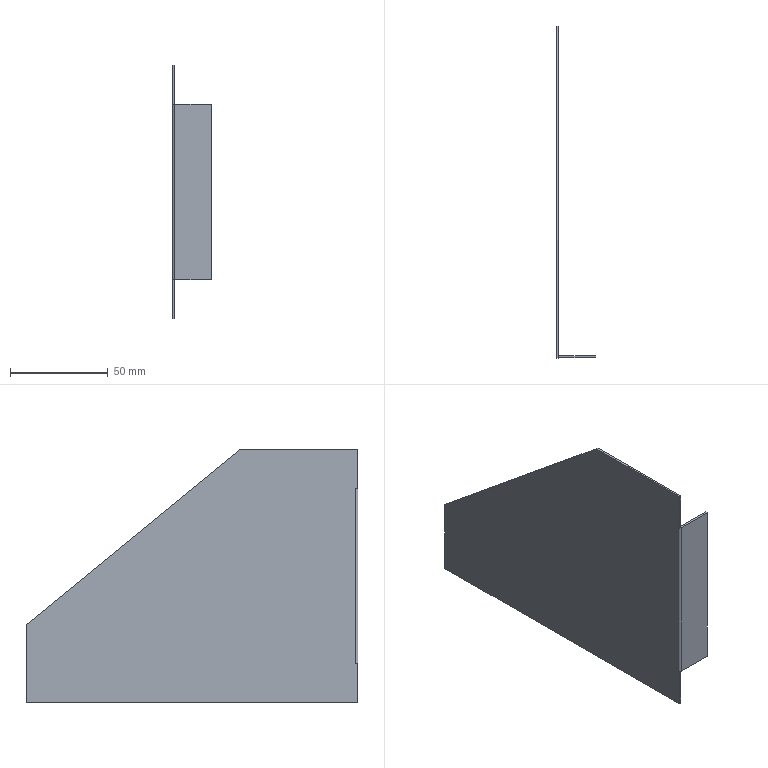Component | SolidWorks | WeldmentDrawing-1_AirDuct2-1 | 1 solid | 19 faces | volume 18837 mm3 | plane 17 | cylinder 2 | commonest cylinder face diameters 2.2 x1 0.2 x1